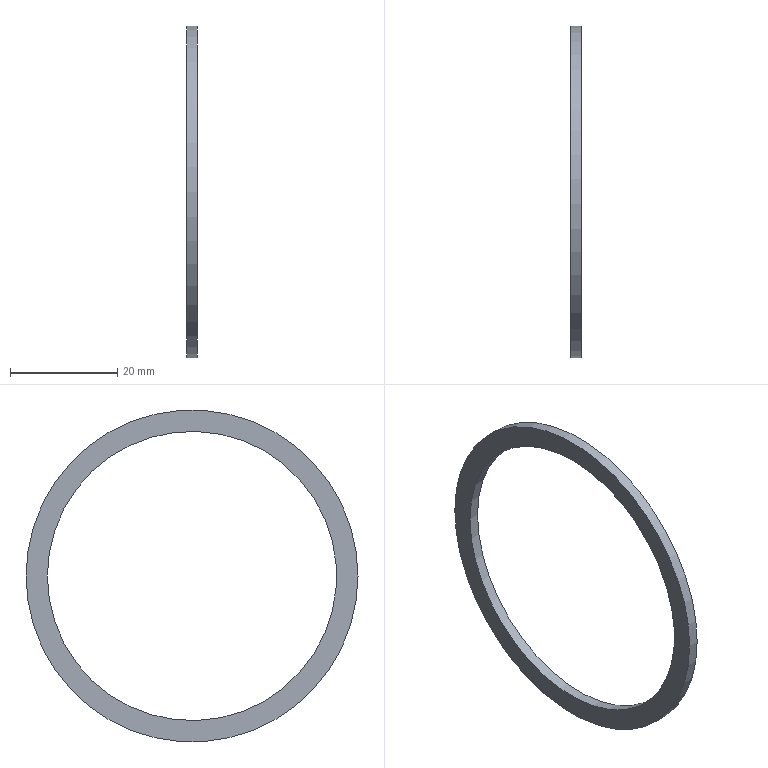Component | NX | DATIAOZHENGHUAN | 1 solid | 4 faces | box 2 x 62 x 62 mm | volume 1458 mm3 | cylinder 2 | plane 2 | commonest cylinder face diameters 62 x1 54 x1
STEP:
#1=CARTESIAN_POINT('',(0.,0.,0.));
#2=DIRECTION('',(0.,0.,1.));
#3=DIRECTION('',(1.,0.,0.));
#4=AXIS2_PLACEMENT_3D('',#1,#2,#3);
#5=CARTESIAN_POINT('',(101.,231.,-88.));
#6=VERTEX_POINT('',#5);
#7=CARTESIAN_POINT('',(101.,200.,-88.));
#8=DIRECTION('',(1.,0.,0.));
#9=DIRECTION('',(0.,1.,0.));
#10=AXIS2_PLACEMENT_3D('',#7,#8,#9);
#11=CIRCLE('',#10,31.);
#12=CARTESIAN_POINT('',(101.,200.,-88.));
#13=DIRECTION('',(-1.,0.,0.));
#14=DIRECTION('',(0.,0.,1.));
#15=AXIS2_PLACEMENT_3D('',#12,#13,#14);
#16=CYLINDRICAL_SURFACE('',#15,31.);
#17=CARTESIAN_POINT('',(7.854,0.));
#18=DIRECTION('',(-1.,0.));
#19=VECTOR('',#18,1.);
#20=LINE('',#17,#19);
#21=(GEOMETRIC_REPRESENTATION_CONTEXT(2)PARAMETRIC_REPRESENTATION_CONTEXT()REPRESENTATION_CONTEXT('',''));
#22=DEFINITIONAL_REPRESENTATION('',(#20),#21);
#23=PCURVE('',#16,#22);
#24=CARTESIAN_POINT('',(101.,200.,-88.));
#25=DIRECTION('',(1.,0.,0.));
#26=DIRECTION('',(0.,0.,-1.));
#27=AXIS2_PLACEMENT_3D('',#24,#25,#26);
#28=PLANE('',#27);
#29=CARTESIAN_POINT('',(0.,0.));
#30=DIRECTION('',(0.,1.));
#31=AXIS2_PLACEMENT_2D('',#29,#30);
#32=CIRCLE('',#31,31.);
#33=(GEOMETRIC_REPRESENTATION_CONTEXT(2)PARAMETRIC_REPRESENTATION_CONTEXT()REPRESENTATION_CONTEXT('',''));
#34=DEFINITIONAL_REPRESENTATION('',(#32),#33);
#35=PCURVE('',#28,#34);
#36=SURFACE_CURVE('',#11,(#23,#35),.PCURVE_S1.);
#37=EDGE_CURVE('',#6,#6,#36,.T.);
#38=ORIENTED_EDGE('',*,*,#37,.F.);
#39=CARTESIAN_POINT('',(99.,231.,-88.));
#40=VERTEX_POINT('',#39);
#41=CARTESIAN_POINT('',(101.,231.,-88.));
#42=CARTESIAN_POINT('',(99.,231.,-88.));
#43=B_SPLINE_CURVE_WITH_KNOTS('',1,(#41,#42),.UNSPECIFIED.,.F.,.F.,(2,2),(0.,2.),.PIECEWISE_BEZIER_KNOTS.);
#44=CARTESIAN_POINT('',(7.854,0.));
#45=DIRECTION('',(0.,1.));
#46=VECTOR('',#45,1.);
#47=LINE('',#44,#46);
#48=(GEOMETRIC_REPRESENTATION_CONTEXT(2)PARAMETRIC_REPRESENTATION_CONTEXT()REPRESENTATION_CONTEXT('',''));
#49=DEFINITIONAL_REPRESENTATION('',(#47),#48);
#50=PCURVE('',#16,#49);
#51=CARTESIAN_POINT('',(1.571,0.));
#52=DIRECTION('',(0.,1.));
#53=VECTOR('',#52,1.);
#54=LINE('',#51,#53);
#55=(GEOMETRIC_REPRESENTATION_CONTEXT(2)PARAMETRIC_REPRESENTATION_CONTEXT()REPRESENTATION_CONTEXT('',''));
#56=DEFINITIONAL_REPRESENTATION('',(#54),#55);
#57=PCURVE('',#16,#56);
#58=SEAM_CURVE('',#43,(#50,#57),.PCURVE_S1.);
#59=EDGE_CURVE('',#6,#40,#58,.T.);
#60=ORIENTED_EDGE('',*,*,#59,.T.);
#61=CARTESIAN_POINT('',(99.,200.,-88.));
#62=DIRECTION('',(1.,0.,0.));
#63=DIRECTION('',(0.,1.,0.));
#64=AXIS2_PLACEMENT_3D('',#61,#62,#63);
#65=CIRCLE('',#64,31.);
#66=CARTESIAN_POINT('',(7.854,2.));
#67=DIRECTION('',(-1.,0.));
#68=VECTOR('',#67,1.);
#69=LINE('',#66,#68);
#70=(GEOMETRIC_REPRESENTATION_CONTEXT(2)PARAMETRIC_REPRESENTATION_CONTEXT()REPRESENTATION_CONTEXT('',''));
#71=DEFINITIONAL_REPRESENTATION('',(#69),#70);
#72=PCURVE('',#16,#71);
#73=CARTESIAN_POINT('',(99.,200.,-88.));
#74=DIRECTION('',(1.,0.,0.));
#75=DIRECTION('',(0.,0.,-1.));
#76=AXIS2_PLACEMENT_3D('',#73,#74,#75);
#77=PLANE('',#76);
#78=CARTESIAN_POINT('',(0.,0.));
#79=DIRECTION('',(0.,1.));
#80=AXIS2_PLACEMENT_2D('',#78,#79);
#81=CIRCLE('',#80,31.);
#82=(GEOMETRIC_REPRESENTATION_CONTEXT(2)PARAMETRIC_REPRESENTATION_CONTEXT()REPRESENTATION_CONTEXT('',''));
#83=DEFINITIONAL_REPRESENTATION('',(#81),#82);
#84=PCURVE('',#77,#83);
#85=SURFACE_CURVE('',#65,(#72,#84),.PCURVE_S1.);
#86=EDGE_CURVE('',#40,#40,#85,.T.);
#87=ORIENTED_EDGE('',*,*,#86,.T.);
#88=ORIENTED_EDGE('',*,*,#59,.F.);
#89=EDGE_LOOP('',(#38,#60,#87,#88));
#90=FACE_BOUND('',#89,.T.);
#91=ADVANCED_FACE('',(#90),#16,.T.);
#92=CARTESIAN_POINT('',(101.,227.,-88.));
#93=VERTEX_POINT('',#92);
#94=CARTESIAN_POINT('',(101.,200.,-88.));
#95=DIRECTION('',(1.,0.,0.));
#96=DIRECTION('',(0.,1.,0.));
#97=AXIS2_PLACEMENT_3D('',#94,#95,#96);
#98=CIRCLE('',#97,27.);
#99=CARTESIAN_POINT('',(101.,200.,-88.));
#100=DIRECTION('',(-1.,0.,0.));
#101=DIRECTION('',(0.,0.,1.));
#102=AXIS2_PLACEMENT_3D('',#99,#100,#101);
#103=CYLINDRICAL_SURFACE('',#102,27.);
#104=CARTESIAN_POINT('',(7.854,0.));
#105=DIRECTION('',(-1.,0.));
#106=VECTOR('',#105,1.);
#107=LINE('',#104,#106);
#108=(GEOMETRIC_REPRESENTATION_CONTEXT(2)PARAMETRIC_REPRESENTATION_CONTEXT()REPRESENTATION_CONTEXT('',''));
#109=DEFINITIONAL_REPRESENTATION('',(#107),#108);
#110=PCURVE('',#103,#109);
#111=CARTESIAN_POINT('',(0.,0.));
#112=DIRECTION('',(0.,1.));
#113=AXIS2_PLACEMENT_2D('',#111,#112);
#114=CIRCLE('',#113,27.);
#115=(GEOMETRIC_REPRESENTATION_CONTEXT(2)PARAMETRIC_REPRESENTATION_CONTEXT()REPRESENTATION_CONTEXT('',''));
#116=DEFINITIONAL_REPRESENTATION('',(#114),#115);
#117=PCURVE('',#28,#116);
#118=SURFACE_CURVE('',#98,(#110,#117),.PCURVE_S1.);
#119=EDGE_CURVE('',#93,#93,#118,.T.);
#120=ORIENTED_EDGE('',*,*,#119,.F.);
#121=CARTESIAN_POINT('',(99.,227.,-88.));
#122=VERTEX_POINT('',#121);
#123=CARTESIAN_POINT('',(101.,227.,-88.));
#124=CARTESIAN_POINT('',(99.,227.,-88.));
#125=B_SPLINE_CURVE_WITH_KNOTS('',1,(#123,#124),.UNSPECIFIED.,.F.,.F.,(2,2),(0.,2.),.PIECEWISE_BEZIER_KNOTS.);
#126=CARTESIAN_POINT('',(7.854,0.));
#127=DIRECTION('',(0.,1.));
#128=VECTOR('',#127,1.);
#129=LINE('',#126,#128);
#130=(GEOMETRIC_REPRESENTATION_CONTEXT(2)PARAMETRIC_REPRESENTATION_CONTEXT()REPRESENTATION_CONTEXT('',''));
#131=DEFINITIONAL_REPRESENTATION('',(#129),#130);
#132=PCURVE('',#103,#131);
#133=CARTESIAN_POINT('',(1.571,0.));
#134=DIRECTION('',(0.,1.));
#135=VECTOR('',#134,1.);
#136=LINE('',#133,#135);
#137=(GEOMETRIC_REPRESENTATION_CONTEXT(2)PARAMETRIC_REPRESENTATION_CONTEXT()REPRESENTATION_CONTEXT('',''));
#138=DEFINITIONAL_REPRESENTATION('',(#136),#137);
#139=PCURVE('',#103,#138);
#140=SEAM_CURVE('',#125,(#132,#139),.PCURVE_S1.);
#141=EDGE_CURVE('',#93,#122,#140,.T.);
#142=ORIENTED_EDGE('',*,*,#141,.T.);
#143=CARTESIAN_POINT('',(99.,200.,-88.));
#144=DIRECTION('',(1.,0.,0.));
#145=DIRECTION('',(0.,1.,0.));
#146=AXIS2_PLACEMENT_3D('',#143,#144,#145);
#147=CIRCLE('',#146,27.);
#148=CARTESIAN_POINT('',(7.854,2.));
#149=DIRECTION('',(-1.,0.));
#150=VECTOR('',#149,1.);
#151=LINE('',#148,#150);
#152=(GEOMETRIC_REPRESENTATION_CONTEXT(2)PARAMETRIC_REPRESENTATION_CONTEXT()REPRESENTATION_CONTEXT('',''));
#153=DEFINITIONAL_REPRESENTATION('',(#151),#152);
#154=PCURVE('',#103,#153);
#155=CARTESIAN_POINT('',(0.,0.));
#156=DIRECTION('',(0.,1.));
#157=AXIS2_PLACEMENT_2D('',#155,#156);
#158=CIRCLE('',#157,27.);
#159=(GEOMETRIC_REPRESENTATION_CONTEXT(2)PARAMETRIC_REPRESENTATION_CONTEXT()REPRESENTATION_CONTEXT('',''));
#160=DEFINITIONAL_REPRESENTATION('',(#158),#159);
#161=PCURVE('',#77,#160);
#162=SURFACE_CURVE('',#147,(#154,#161),.PCURVE_S1.);
#163=EDGE_CURVE('',#122,#122,#162,.T.);
#164=ORIENTED_EDGE('',*,*,#163,.T.);
#165=ORIENTED_EDGE('',*,*,#141,.F.);
#166=EDGE_LOOP('',(#120,#142,#164,#165));
#167=FACE_BOUND('',#166,.F.);
#168=ADVANCED_FACE('',(#167),#103,.F.);
#169=ORIENTED_EDGE('',*,*,#37,.T.);
#170=EDGE_LOOP('',(#169));
#171=FACE_BOUND('',#170,.T.);
#172=ORIENTED_EDGE('',*,*,#119,.F.);
#173=EDGE_LOOP('',(#172));
#174=FACE_BOUND('',#173,.T.);
#175=ADVANCED_FACE('',(#171,#174),#28,.T.);
#176=ORIENTED_EDGE('',*,*,#86,.F.);
#177=EDGE_LOOP('',(#176));
#178=FACE_BOUND('',#177,.T.);
#179=ORIENTED_EDGE('',*,*,#163,.T.);
#180=EDGE_LOOP('',(#179));
#181=FACE_BOUND('',#180,.T.);
#182=ADVANCED_FACE('',(#178,#181),#77,.F.);
#183=CLOSED_SHELL('',(#91,#168,#175,#182));
#184=MANIFOLD_SOLID_BREP('',#183);
#185=(LENGTH_UNIT()NAMED_UNIT(*)SI_UNIT(.MILLI.,.METRE.));
#186=UNCERTAINTY_MEASURE_WITH_UNIT(LENGTH_MEASURE(0.00001),#185,'','');
#187=(NAMED_UNIT(*)PLANE_ANGLE_UNIT()SI_UNIT($,.RADIAN.));
#188=(NAMED_UNIT(*)SI_UNIT($,.STERADIAN.)SOLID_ANGLE_UNIT());
#189=(GEOMETRIC_REPRESENTATION_CONTEXT(3)GLOBAL_UNCERTAINTY_ASSIGNED_CONTEXT((#186))GLOBAL_UNIT_ASSIGNED_CONTEXT((#185,#187,#188))REPRESENTATION_CONTEXT('',''));
#190=ADVANCED_BREP_SHAPE_REPRESENTATION('',(#4,#184),#189);